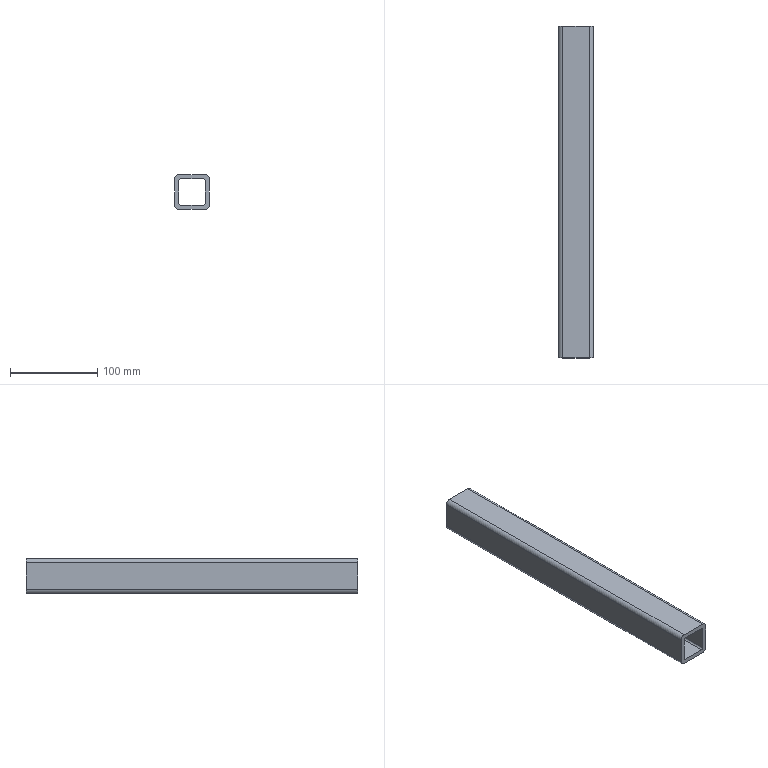Component | SolidWorks | 40-40SquareTube7-1 | 1 solid | 18 faces | box 40 x 380 x 40 mm | volume 259150 mm3 | plane 10 | cylinder 8 | commonest cylinder face diameters 10 x4 4 x4
build123d program:
from build123d import *

# Parameters (mm, degrees)
BOSS_EXTRUDE1_DEPTH = 190


with BuildPart() as part:
    # Sketch1 → Boss-Extrude1 (new, symmetric)
    with BuildSketch(Plane.XY):
        with BuildLine():
            Line((-15, -20), (15, -20))
            ThreePointArc((15, -20), (18.536, -18.536), (20, -15))
            Line((20, -15), (20, 15))
            ThreePointArc((20, 15), (18.536, 18.536), (15, 20))
            Line((15, 20), (-15, 20))
            ThreePointArc((-15, 20), (-18.536, 18.536), (-20, 15))
            Line((-20, 15), (-20, -15))
            ThreePointArc((-20, -15), (-18.536, -18.536), (-15, -20))
        make_face()
        with BuildLine():
            Line((-13, -15), (13, -15))
            ThreePointArc((13, -15), (14.414, -14.414), (15, -13))
            Line((15, -13), (15, 13))
            ThreePointArc((15, 13), (14.414, 14.414), (13, 15))
            Line((13, 15), (-13, 15))
            ThreePointArc((-13, 15), (-14.414, 14.414), (-15, 13))
            Line((-15, 13), (-15, -13))
            ThreePointArc((-15, -13), (-14.414, -14.414), (-13, -15))
        make_face(mode=Mode.SUBTRACT)
    extrude(amount=BOSS_EXTRUDE1_DEPTH, both=True)


solid = part.part

# Placed as in the assembly
solid = solid.moved(Location((17.398, 237.837, 160), (90, 0, 0)))
STEP:
#1=CARTESIAN_POINT('',(1.472,16.844,5.709));
#2=VERTEX_POINT('',#1);
#3=CARTESIAN_POINT('',(1.276,16.844,5.512));
#4=VERTEX_POINT('',#3);
#5=CARTESIAN_POINT('',(1.276,16.844,5.709));
#6=DIRECTION('',(0.,1.,0.));
#7=DIRECTION('',(0.,0.,-1.));
#8=AXIS2_PLACEMENT_3D('',#5,#6,#7);
#9=CIRCLE('',#8,0.1969);
#10=EDGE_CURVE('',#2,#4,#9,.T.);
#11=ORIENTED_EDGE('',*,*,#10,.T.);
#12=CARTESIAN_POINT('',(0.09441,16.844,5.512));
#13=VERTEX_POINT('',#12);
#14=CARTESIAN_POINT('',(1.276,16.844,5.512));
#15=DIRECTION('',(-1.,0.,0.));
#16=VECTOR('',#15,39.37);
#17=LINE('',#14,#16);
#18=EDGE_CURVE('',#4,#13,#17,.T.);
#19=ORIENTED_EDGE('',*,*,#18,.T.);
#20=CARTESIAN_POINT('',(-0.1024,16.844,5.709));
#21=VERTEX_POINT('',#20);
#22=CARTESIAN_POINT('',(0.09441,16.844,5.709));
#23=DIRECTION('',(0.,1.,0.));
#24=DIRECTION('',(0.,0.,1.));
#25=AXIS2_PLACEMENT_3D('',#22,#23,#24);
#26=CIRCLE('',#25,0.1969);
#27=EDGE_CURVE('',#13,#21,#26,.T.);
#28=ORIENTED_EDGE('',*,*,#27,.T.);
#29=CARTESIAN_POINT('',(-0.1024,16.844,6.89));
#30=VERTEX_POINT('',#29);
#31=CARTESIAN_POINT('',(-0.1024,16.844,6.89));
#32=DIRECTION('',(0.,-0.,1.));
#33=VECTOR('',#32,39.37);
#34=LINE('',#31,#33);
#35=EDGE_CURVE('',#21,#30,#34,.T.);
#36=ORIENTED_EDGE('',*,*,#35,.T.);
#37=CARTESIAN_POINT('',(0.09441,16.844,7.087));
#38=VERTEX_POINT('',#37);
#39=CARTESIAN_POINT('',(0.09441,16.844,6.89));
#40=DIRECTION('',(0.,1.,0.));
#41=DIRECTION('',(0.,0.,1.));
#42=AXIS2_PLACEMENT_3D('',#39,#40,#41);
#43=CIRCLE('',#42,0.1969);
#44=EDGE_CURVE('',#30,#38,#43,.T.);
#45=ORIENTED_EDGE('',*,*,#44,.T.);
#46=CARTESIAN_POINT('',(1.276,16.844,7.087));
#47=VERTEX_POINT('',#46);
#48=CARTESIAN_POINT('',(1.276,16.844,7.087));
#49=DIRECTION('',(1.,-0.,0.));
#50=VECTOR('',#49,39.37);
#51=LINE('',#48,#50);
#52=EDGE_CURVE('',#38,#47,#51,.T.);
#53=ORIENTED_EDGE('',*,*,#52,.T.);
#54=CARTESIAN_POINT('',(1.472,16.844,6.89));
#55=VERTEX_POINT('',#54);
#56=CARTESIAN_POINT('',(1.276,16.844,6.89));
#57=DIRECTION('',(0.,1.,0.));
#58=DIRECTION('',(0.,0.,1.));
#59=AXIS2_PLACEMENT_3D('',#56,#57,#58);
#60=CIRCLE('',#59,0.1969);
#61=EDGE_CURVE('',#47,#55,#60,.T.);
#62=ORIENTED_EDGE('',*,*,#61,.T.);
#63=CARTESIAN_POINT('',(1.472,16.844,6.89));
#64=DIRECTION('',(0.,0.,-1.));
#65=VECTOR('',#64,39.37);
#66=LINE('',#63,#65);
#67=EDGE_CURVE('',#55,#2,#66,.T.);
#68=ORIENTED_EDGE('',*,*,#67,.T.);
#69=EDGE_LOOP('',(#11,#19,#28,#36,#45,#53,#62,#68));
#70=FACE_OUTER_BOUND('',#69,.T.);
#71=CARTESIAN_POINT('',(1.197,16.844,5.709));
#72=VERTEX_POINT('',#71);
#73=CARTESIAN_POINT('',(0.1732,16.844,5.709));
#74=VERTEX_POINT('',#73);
#75=CARTESIAN_POINT('',(1.197,16.844,5.709));
#76=DIRECTION('',(-1.,0.,0.));
#77=VECTOR('',#76,39.37);
#78=LINE('',#75,#77);
#79=EDGE_CURVE('',#72,#74,#78,.T.);
#80=ORIENTED_EDGE('',*,*,#79,.F.);
#81=CARTESIAN_POINT('',(1.276,16.844,5.787));
#82=VERTEX_POINT('',#81);
#83=CARTESIAN_POINT('',(1.197,16.844,5.787));
#84=DIRECTION('',(0.,1.,0.));
#85=DIRECTION('',(0.,0.,-1.));
#86=AXIS2_PLACEMENT_3D('',#83,#84,#85);
#87=CIRCLE('',#86,0.07874);
#88=EDGE_CURVE('',#82,#72,#87,.T.);
#89=ORIENTED_EDGE('',*,*,#88,.F.);
#90=CARTESIAN_POINT('',(1.276,16.844,6.811));
#91=VERTEX_POINT('',#90);
#92=CARTESIAN_POINT('',(1.276,16.844,6.811));
#93=DIRECTION('',(0.,0.,-1.));
#94=VECTOR('',#93,39.37);
#95=LINE('',#92,#94);
#96=EDGE_CURVE('',#91,#82,#95,.T.);
#97=ORIENTED_EDGE('',*,*,#96,.F.);
#98=CARTESIAN_POINT('',(1.197,16.844,6.89));
#99=VERTEX_POINT('',#98);
#100=CARTESIAN_POINT('',(1.197,16.844,6.811));
#101=DIRECTION('',(0.,1.,0.));
#102=DIRECTION('',(0.,0.,1.));
#103=AXIS2_PLACEMENT_3D('',#100,#101,#102);
#104=CIRCLE('',#103,0.07874);
#105=EDGE_CURVE('',#99,#91,#104,.T.);
#106=ORIENTED_EDGE('',*,*,#105,.F.);
#107=CARTESIAN_POINT('',(0.1732,16.844,6.89));
#108=VERTEX_POINT('',#107);
#109=CARTESIAN_POINT('',(1.197,16.844,6.89));
#110=DIRECTION('',(1.,-0.,-0.));
#111=VECTOR('',#110,39.37);
#112=LINE('',#109,#111);
#113=EDGE_CURVE('',#108,#99,#112,.T.);
#114=ORIENTED_EDGE('',*,*,#113,.F.);
#115=CARTESIAN_POINT('',(0.09441,16.844,6.811));
#116=VERTEX_POINT('',#115);
#117=CARTESIAN_POINT('',(0.1732,16.844,6.811));
#118=DIRECTION('',(0.,1.,0.));
#119=DIRECTION('',(0.,0.,1.));
#120=AXIS2_PLACEMENT_3D('',#117,#118,#119);
#121=CIRCLE('',#120,0.07874);
#122=EDGE_CURVE('',#116,#108,#121,.T.);
#123=ORIENTED_EDGE('',*,*,#122,.F.);
#124=CARTESIAN_POINT('',(0.09441,16.844,5.787));
#125=VERTEX_POINT('',#124);
#126=CARTESIAN_POINT('',(0.09441,16.844,6.811));
#127=DIRECTION('',(0.,-0.,1.));
#128=VECTOR('',#127,39.37);
#129=LINE('',#126,#128);
#130=EDGE_CURVE('',#125,#116,#129,.T.);
#131=ORIENTED_EDGE('',*,*,#130,.F.);
#132=CARTESIAN_POINT('',(0.1732,16.844,5.787));
#133=DIRECTION('',(0.,1.,0.));
#134=DIRECTION('',(0.,0.,1.));
#135=AXIS2_PLACEMENT_3D('',#132,#133,#134);
#136=CIRCLE('',#135,0.07874);
#137=EDGE_CURVE('',#74,#125,#136,.T.);
#138=ORIENTED_EDGE('',*,*,#137,.F.);
#139=EDGE_LOOP('',(#80,#89,#97,#106,#114,#123,#131,#138));
#140=FACE_BOUND('',#139,.T.);
#141=CARTESIAN_POINT('',(1.276,16.844,5.709));
#142=DIRECTION('',(0.,1.,0.));
#143=DIRECTION('',(0.,0.,-1.));
#144=AXIS2_PLACEMENT_3D('',#141,#142,#143);
#145=PLANE('',#144);
#146=ADVANCED_FACE('',(#70,#140),#145,.T.);
#147=CARTESIAN_POINT('',(1.472,1.883,5.709));
#148=VERTEX_POINT('',#147);
#149=CARTESIAN_POINT('',(1.276,1.883,5.512));
#150=VERTEX_POINT('',#149);
#151=CARTESIAN_POINT('',(1.276,1.883,5.709));
#152=DIRECTION('',(0.,1.,0.));
#153=DIRECTION('',(0.,0.,-1.));
#154=AXIS2_PLACEMENT_3D('',#151,#152,#153);
#155=CIRCLE('',#154,0.1969);
#156=EDGE_CURVE('',#148,#150,#155,.T.);
#157=ORIENTED_EDGE('',*,*,#156,.F.);
#158=CARTESIAN_POINT('',(1.472,1.883,6.89));
#159=VERTEX_POINT('',#158);
#160=CARTESIAN_POINT('',(1.472,1.883,6.89));
#161=DIRECTION('',(0.,0.,-1.));
#162=VECTOR('',#161,39.37);
#163=LINE('',#160,#162);
#164=EDGE_CURVE('',#159,#148,#163,.T.);
#165=ORIENTED_EDGE('',*,*,#164,.F.);
#166=CARTESIAN_POINT('',(1.276,1.883,7.087));
#167=VERTEX_POINT('',#166);
#168=CARTESIAN_POINT('',(1.276,1.883,6.89));
#169=DIRECTION('',(0.,1.,0.));
#170=DIRECTION('',(0.,0.,1.));
#171=AXIS2_PLACEMENT_3D('',#168,#169,#170);
#172=CIRCLE('',#171,0.1969);
#173=EDGE_CURVE('',#167,#159,#172,.T.);
#174=ORIENTED_EDGE('',*,*,#173,.F.);
#175=CARTESIAN_POINT('',(0.09441,1.883,7.087));
#176=VERTEX_POINT('',#175);
#177=CARTESIAN_POINT('',(1.276,1.883,7.087));
#178=DIRECTION('',(1.,-0.,0.));
#179=VECTOR('',#178,39.37);
#180=LINE('',#177,#179);
#181=EDGE_CURVE('',#176,#167,#180,.T.);
#182=ORIENTED_EDGE('',*,*,#181,.F.);
#183=CARTESIAN_POINT('',(-0.1024,1.883,6.89));
#184=VERTEX_POINT('',#183);
#185=CARTESIAN_POINT('',(0.09441,1.883,6.89));
#186=DIRECTION('',(0.,1.,0.));
#187=DIRECTION('',(0.,0.,1.));
#188=AXIS2_PLACEMENT_3D('',#185,#186,#187);
#189=CIRCLE('',#188,0.1969);
#190=EDGE_CURVE('',#184,#176,#189,.T.);
#191=ORIENTED_EDGE('',*,*,#190,.F.);
#192=CARTESIAN_POINT('',(-0.1024,1.883,5.709));
#193=VERTEX_POINT('',#192);
#194=CARTESIAN_POINT('',(-0.1024,1.883,6.89));
#195=DIRECTION('',(0.,-0.,1.));
#196=VECTOR('',#195,39.37);
#197=LINE('',#194,#196);
#198=EDGE_CURVE('',#193,#184,#197,.T.);
#199=ORIENTED_EDGE('',*,*,#198,.F.);
#200=CARTESIAN_POINT('',(0.09441,1.883,5.512));
#201=VERTEX_POINT('',#200);
#202=CARTESIAN_POINT('',(0.09441,1.883,5.709));
#203=DIRECTION('',(0.,1.,0.));
#204=DIRECTION('',(0.,0.,1.));
#205=AXIS2_PLACEMENT_3D('',#202,#203,#204);
#206=CIRCLE('',#205,0.1969);
#207=EDGE_CURVE('',#201,#193,#206,.T.);
#208=ORIENTED_EDGE('',*,*,#207,.F.);
#209=CARTESIAN_POINT('',(1.276,1.883,5.512));
#210=DIRECTION('',(-1.,0.,0.));
#211=VECTOR('',#210,39.37);
#212=LINE('',#209,#211);
#213=EDGE_CURVE('',#150,#201,#212,.T.);
#214=ORIENTED_EDGE('',*,*,#213,.F.);
#215=EDGE_LOOP('',(#157,#165,#174,#182,#191,#199,#208,#214));
#216=FACE_OUTER_BOUND('',#215,.T.);
#217=CARTESIAN_POINT('',(1.276,1.883,5.787));
#218=VERTEX_POINT('',#217);
#219=CARTESIAN_POINT('',(1.197,1.883,5.709));
#220=VERTEX_POINT('',#219);
#221=CARTESIAN_POINT('',(1.197,1.883,5.787));
#222=DIRECTION('',(0.,1.,0.));
#223=DIRECTION('',(0.,0.,-1.));
#224=AXIS2_PLACEMENT_3D('',#221,#222,#223);
#225=CIRCLE('',#224,0.07874);
#226=EDGE_CURVE('',#218,#220,#225,.T.);
#227=ORIENTED_EDGE('',*,*,#226,.T.);
#228=CARTESIAN_POINT('',(0.1732,1.883,5.709));
#229=VERTEX_POINT('',#228);
#230=CARTESIAN_POINT('',(1.197,1.883,5.709));
#231=DIRECTION('',(-1.,0.,0.));
#232=VECTOR('',#231,39.37);
#233=LINE('',#230,#232);
#234=EDGE_CURVE('',#220,#229,#233,.T.);
#235=ORIENTED_EDGE('',*,*,#234,.T.);
#236=CARTESIAN_POINT('',(0.09441,1.883,5.787));
#237=VERTEX_POINT('',#236);
#238=CARTESIAN_POINT('',(0.1732,1.883,5.787));
#239=DIRECTION('',(0.,1.,0.));
#240=DIRECTION('',(0.,0.,1.));
#241=AXIS2_PLACEMENT_3D('',#238,#239,#240);
#242=CIRCLE('',#241,0.07874);
#243=EDGE_CURVE('',#229,#237,#242,.T.);
#244=ORIENTED_EDGE('',*,*,#243,.T.);
#245=CARTESIAN_POINT('',(0.09441,1.883,6.811));
#246=VERTEX_POINT('',#245);
#247=CARTESIAN_POINT('',(0.09441,1.883,6.811));
#248=DIRECTION('',(0.,-0.,1.));
#249=VECTOR('',#248,39.37);
#250=LINE('',#247,#249);
#251=EDGE_CURVE('',#237,#246,#250,.T.);
#252=ORIENTED_EDGE('',*,*,#251,.T.);
#253=CARTESIAN_POINT('',(0.1732,1.883,6.89));
#254=VERTEX_POINT('',#253);
#255=CARTESIAN_POINT('',(0.1732,1.883,6.811));
#256=DIRECTION('',(0.,1.,0.));
#257=DIRECTION('',(0.,0.,1.));
#258=AXIS2_PLACEMENT_3D('',#255,#256,#257);
#259=CIRCLE('',#258,0.07874);
#260=EDGE_CURVE('',#246,#254,#259,.T.);
#261=ORIENTED_EDGE('',*,*,#260,.T.);
#262=CARTESIAN_POINT('',(1.197,1.883,6.89));
#263=VERTEX_POINT('',#262);
#264=CARTESIAN_POINT('',(1.197,1.883,6.89));
#265=DIRECTION('',(1.,-0.,-0.));
#266=VECTOR('',#265,39.37);
#267=LINE('',#264,#266);
#268=EDGE_CURVE('',#254,#263,#267,.T.);
#269=ORIENTED_EDGE('',*,*,#268,.T.);
#270=CARTESIAN_POINT('',(1.276,1.883,6.811));
#271=VERTEX_POINT('',#270);
#272=CARTESIAN_POINT('',(1.197,1.883,6.811));
#273=DIRECTION('',(0.,1.,0.));
#274=DIRECTION('',(0.,0.,1.));
#275=AXIS2_PLACEMENT_3D('',#272,#273,#274);
#276=CIRCLE('',#275,0.07874);
#277=EDGE_CURVE('',#263,#271,#276,.T.);
#278=ORIENTED_EDGE('',*,*,#277,.T.);
#279=CARTESIAN_POINT('',(1.276,1.883,6.811));
#280=DIRECTION('',(0.,0.,-1.));
#281=VECTOR('',#280,39.37);
#282=LINE('',#279,#281);
#283=EDGE_CURVE('',#271,#218,#282,.T.);
#284=ORIENTED_EDGE('',*,*,#283,.T.);
#285=EDGE_LOOP('',(#227,#235,#244,#252,#261,#269,#278,#284));
#286=FACE_BOUND('',#285,.T.);
#287=CARTESIAN_POINT('',(1.276,1.883,5.709));
#288=DIRECTION('',(0.,1.,0.));
#289=DIRECTION('',(0.,0.,-1.));
#290=AXIS2_PLACEMENT_3D('',#287,#288,#289);
#291=PLANE('',#290);
#292=ADVANCED_FACE('',(#216,#286),#291,.F.);
#293=ORIENTED_EDGE('',*,*,#156,.T.);
#294=CARTESIAN_POINT('',(1.276,16.844,5.512));
#295=DIRECTION('',(-0.,-1.,-0.));
#296=VECTOR('',#295,39.37);
#297=LINE('',#294,#296);
#298=EDGE_CURVE('',#4,#150,#297,.T.);
#299=ORIENTED_EDGE('',*,*,#298,.F.);
#300=ORIENTED_EDGE('',*,*,#10,.F.);
#301=CARTESIAN_POINT('',(1.472,16.844,5.709));
#302=DIRECTION('',(-0.,-1.,-0.));
#303=VECTOR('',#302,39.37);
#304=LINE('',#301,#303);
#305=EDGE_CURVE('',#2,#148,#304,.T.);
#306=ORIENTED_EDGE('',*,*,#305,.T.);
#307=EDGE_LOOP('',(#293,#299,#300,#306));
#308=FACE_OUTER_BOUND('',#307,.T.);
#309=CARTESIAN_POINT('',(1.276,16.844,5.709));
#310=DIRECTION('',(-0.,-1.,-0.));
#311=DIRECTION('',(0.,0.,1.));
#312=AXIS2_PLACEMENT_3D('',#309,#310,#311);
#313=CYLINDRICAL_SURFACE('',#312,0.1969);
#314=ADVANCED_FACE('',(#308),#313,.T.);
#315=ORIENTED_EDGE('',*,*,#213,.T.);
#316=CARTESIAN_POINT('',(0.09441,16.844,5.512));
#317=DIRECTION('',(-0.,-1.,-0.));
#318=VECTOR('',#317,39.37);
#319=LINE('',#316,#318);
#320=EDGE_CURVE('',#13,#201,#319,.T.);
#321=ORIENTED_EDGE('',*,*,#320,.F.);
#322=ORIENTED_EDGE('',*,*,#18,.F.);
#323=ORIENTED_EDGE('',*,*,#298,.T.);
#324=EDGE_LOOP('',(#315,#321,#322,#323));
#325=FACE_OUTER_BOUND('',#324,.T.);
#326=CARTESIAN_POINT('',(1.276,16.844,5.512));
#327=DIRECTION('',(0.,-0.,1.));
#328=DIRECTION('',(0.,1.,0.));
#329=AXIS2_PLACEMENT_3D('',#326,#327,#328);
#330=PLANE('',#329);
#331=ADVANCED_FACE('',(#325),#330,.F.);
#332=ORIENTED_EDGE('',*,*,#207,.T.);
#333=CARTESIAN_POINT('',(-0.1024,16.844,5.709));
#334=DIRECTION('',(-0.,-1.,-0.));
#335=VECTOR('',#334,39.37);
#336=LINE('',#333,#335);
#337=EDGE_CURVE('',#21,#193,#336,.T.);
#338=ORIENTED_EDGE('',*,*,#337,.F.);
#339=ORIENTED_EDGE('',*,*,#27,.F.);
#340=ORIENTED_EDGE('',*,*,#320,.T.);
#341=EDGE_LOOP('',(#332,#338,#339,#340));
#342=FACE_OUTER_BOUND('',#341,.T.);
#343=CARTESIAN_POINT('',(0.09441,16.844,5.709));
#344=DIRECTION('',(-0.,-1.,-0.));
#345=DIRECTION('',(0.,0.,1.));
#346=AXIS2_PLACEMENT_3D('',#343,#344,#345);
#347=CYLINDRICAL_SURFACE('',#346,0.1969);
#348=ADVANCED_FACE('',(#342),#347,.T.);
#349=ORIENTED_EDGE('',*,*,#198,.T.);
#350=CARTESIAN_POINT('',(-0.1024,16.844,6.89));
#351=DIRECTION('',(-0.,-1.,-0.));
#352=VECTOR('',#351,39.37);
#353=LINE('',#350,#352);
#354=EDGE_CURVE('',#30,#184,#353,.T.);
#355=ORIENTED_EDGE('',*,*,#354,.F.);
#356=ORIENTED_EDGE('',*,*,#35,.F.);
#357=ORIENTED_EDGE('',*,*,#337,.T.);
#358=EDGE_LOOP('',(#349,#355,#356,#357));
#359=FACE_OUTER_BOUND('',#358,.T.);
#360=CARTESIAN_POINT('',(-0.1024,16.844,6.89));
#361=DIRECTION('',(1.,-0.,-0.));
#362=DIRECTION('',(-0.,-1.,-0.));
#363=AXIS2_PLACEMENT_3D('',#360,#361,#362);
#364=PLANE('',#363);
#365=ADVANCED_FACE('',(#359),#364,.F.);
#366=ORIENTED_EDGE('',*,*,#190,.T.);
#367=CARTESIAN_POINT('',(0.09441,16.844,7.087));
#368=DIRECTION('',(-0.,-1.,-0.));
#369=VECTOR('',#368,39.37);
#370=LINE('',#367,#369);
#371=EDGE_CURVE('',#38,#176,#370,.T.);
#372=ORIENTED_EDGE('',*,*,#371,.F.);
#373=ORIENTED_EDGE('',*,*,#44,.F.);
#374=ORIENTED_EDGE('',*,*,#354,.T.);
#375=EDGE_LOOP('',(#366,#372,#373,#374));
#376=FACE_OUTER_BOUND('',#375,.T.);
#377=CARTESIAN_POINT('',(0.09441,16.844,6.89));
#378=DIRECTION('',(-0.,-1.,-0.));
#379=DIRECTION('',(0.,0.,1.));
#380=AXIS2_PLACEMENT_3D('',#377,#378,#379);
#381=CYLINDRICAL_SURFACE('',#380,0.1969);
#382=ADVANCED_FACE('',(#376),#381,.T.);
#383=ORIENTED_EDGE('',*,*,#181,.T.);
#384=CARTESIAN_POINT('',(1.276,16.844,7.087));
#385=DIRECTION('',(-0.,-1.,-0.));
#386=VECTOR('',#385,39.37);
#387=LINE('',#384,#386);
#388=EDGE_CURVE('',#47,#167,#387,.T.);
#389=ORIENTED_EDGE('',*,*,#388,.F.);
#390=ORIENTED_EDGE('',*,*,#52,.F.);
#391=ORIENTED_EDGE('',*,*,#371,.T.);
#392=EDGE_LOOP('',(#383,#389,#390,#391));
#393=FACE_OUTER_BOUND('',#392,.T.);
#394=CARTESIAN_POINT('',(1.276,16.844,7.087));
#395=DIRECTION('',(0.,0.,-1.));
#396=DIRECTION('',(-1.,0.,-0.));
#397=AXIS2_PLACEMENT_3D('',#394,#395,#396);
#398=PLANE('',#397);
#399=ADVANCED_FACE('',(#393),#398,.F.);
#400=ORIENTED_EDGE('',*,*,#173,.T.);
#401=CARTESIAN_POINT('',(1.472,16.844,6.89));
#402=DIRECTION('',(-0.,-1.,-0.));
#403=VECTOR('',#402,39.37);
#404=LINE('',#401,#403);
#405=EDGE_CURVE('',#55,#159,#404,.T.);
#406=ORIENTED_EDGE('',*,*,#405,.F.);
#407=ORIENTED_EDGE('',*,*,#61,.F.);
#408=ORIENTED_EDGE('',*,*,#388,.T.);
#409=EDGE_LOOP('',(#400,#406,#407,#408));
#410=FACE_OUTER_BOUND('',#409,.T.);
#411=CARTESIAN_POINT('',(1.276,16.844,6.89));
#412=DIRECTION('',(-0.,-1.,-0.));
#413=DIRECTION('',(0.,0.,1.));
#414=AXIS2_PLACEMENT_3D('',#411,#412,#413);
#415=CYLINDRICAL_SURFACE('',#414,0.1969);
#416=ADVANCED_FACE('',(#410),#415,.T.);
#417=ORIENTED_EDGE('',*,*,#164,.T.);
#418=ORIENTED_EDGE('',*,*,#305,.F.);
#419=ORIENTED_EDGE('',*,*,#67,.F.);
#420=ORIENTED_EDGE('',*,*,#405,.T.);
#421=EDGE_LOOP('',(#417,#418,#419,#420));
#422=FACE_OUTER_BOUND('',#421,.T.);
#423=CARTESIAN_POINT('',(1.472,16.844,6.89));
#424=DIRECTION('',(-1.,0.,0.));
#425=DIRECTION('',(0.,1.,0.));
#426=AXIS2_PLACEMENT_3D('',#423,#424,#425);
#427=PLANE('',#426);
#428=ADVANCED_FACE('',(#422),#427,.F.);
#429=ORIENTED_EDGE('',*,*,#226,.F.);
#430=CARTESIAN_POINT('',(1.276,16.844,5.787));
#431=DIRECTION('',(-0.,-1.,-0.));
#432=VECTOR('',#431,39.37);
#433=LINE('',#430,#432);
#434=EDGE_CURVE('',#82,#218,#433,.T.);
#435=ORIENTED_EDGE('',*,*,#434,.F.);
#436=ORIENTED_EDGE('',*,*,#88,.T.);
#437=CARTESIAN_POINT('',(1.197,16.844,5.709));
#438=DIRECTION('',(-0.,-1.,-0.));
#439=VECTOR('',#438,39.37);
#440=LINE('',#437,#439);
#441=EDGE_CURVE('',#72,#220,#440,.T.);
#442=ORIENTED_EDGE('',*,*,#441,.T.);
#443=EDGE_LOOP('',(#429,#435,#436,#442));
#444=FACE_OUTER_BOUND('',#443,.T.);
#445=CARTESIAN_POINT('',(1.197,16.844,5.787));
#446=DIRECTION('',(-0.,-1.,-0.));
#447=DIRECTION('',(0.,0.,1.));
#448=AXIS2_PLACEMENT_3D('',#445,#446,#447);
#449=CYLINDRICAL_SURFACE('',#448,0.07874);
#450=ADVANCED_FACE('',(#444),#449,.F.);
#451=ORIENTED_EDGE('',*,*,#234,.F.);
#452=ORIENTED_EDGE('',*,*,#441,.F.);
#453=ORIENTED_EDGE('',*,*,#79,.T.);
#454=CARTESIAN_POINT('',(0.1732,16.844,5.709));
#455=DIRECTION('',(-0.,-1.,-0.));
#456=VECTOR('',#455,39.37);
#457=LINE('',#454,#456);
#458=EDGE_CURVE('',#74,#229,#457,.T.);
#459=ORIENTED_EDGE('',*,*,#458,.T.);
#460=EDGE_LOOP('',(#451,#452,#453,#459));
#461=FACE_OUTER_BOUND('',#460,.T.);
#462=CARTESIAN_POINT('',(1.197,16.844,5.709));
#463=DIRECTION('',(0.,-0.,1.));
#464=DIRECTION('',(0.,1.,0.));
#465=AXIS2_PLACEMENT_3D('',#462,#463,#464);
#466=PLANE('',#465);
#467=ADVANCED_FACE('',(#461),#466,.T.);
#468=ORIENTED_EDGE('',*,*,#243,.F.);
#469=ORIENTED_EDGE('',*,*,#458,.F.);
#470=ORIENTED_EDGE('',*,*,#137,.T.);
#471=CARTESIAN_POINT('',(0.09441,16.844,5.787));
#472=DIRECTION('',(-0.,-1.,-0.));
#473=VECTOR('',#472,39.37);
#474=LINE('',#471,#473);
#475=EDGE_CURVE('',#125,#237,#474,.T.);
#476=ORIENTED_EDGE('',*,*,#475,.T.);
#477=EDGE_LOOP('',(#468,#469,#470,#476));
#478=FACE_OUTER_BOUND('',#477,.T.);
#479=CARTESIAN_POINT('',(0.1732,16.844,5.787));
#480=DIRECTION('',(-0.,-1.,-0.));
#481=DIRECTION('',(0.,0.,1.));
#482=AXIS2_PLACEMENT_3D('',#479,#480,#481);
#483=CYLINDRICAL_SURFACE('',#482,0.07874);
#484=ADVANCED_FACE('',(#478),#483,.F.);
#485=ORIENTED_EDGE('',*,*,#251,.F.);
#486=ORIENTED_EDGE('',*,*,#475,.F.);
#487=ORIENTED_EDGE('',*,*,#130,.T.);
#488=CARTESIAN_POINT('',(0.09441,16.844,6.811));
#489=DIRECTION('',(-0.,-1.,-0.));
#490=VECTOR('',#489,39.37);
#491=LINE('',#488,#490);
#492=EDGE_CURVE('',#116,#246,#491,.T.);
#493=ORIENTED_EDGE('',*,*,#492,.T.);
#494=EDGE_LOOP('',(#485,#486,#487,#493));
#495=FACE_OUTER_BOUND('',#494,.T.);
#496=CARTESIAN_POINT('',(0.09441,16.844,6.811));
#497=DIRECTION('',(1.,-0.,-0.));
#498=DIRECTION('',(-0.,-1.,-0.));
#499=AXIS2_PLACEMENT_3D('',#496,#497,#498);
#500=PLANE('',#499);
#501=ADVANCED_FACE('',(#495),#500,.T.);
#502=ORIENTED_EDGE('',*,*,#260,.F.);
#503=ORIENTED_EDGE('',*,*,#492,.F.);
#504=ORIENTED_EDGE('',*,*,#122,.T.);
#505=CARTESIAN_POINT('',(0.1732,16.844,6.89));
#506=DIRECTION('',(-0.,-1.,-0.));
#507=VECTOR('',#506,39.37);
#508=LINE('',#505,#507);
#509=EDGE_CURVE('',#108,#254,#508,.T.);
#510=ORIENTED_EDGE('',*,*,#509,.T.);
#511=EDGE_LOOP('',(#502,#503,#504,#510));
#512=FACE_OUTER_BOUND('',#511,.T.);
#513=CARTESIAN_POINT('',(0.1732,16.844,6.811));
#514=DIRECTION('',(-0.,-1.,-0.));
#515=DIRECTION('',(0.,0.,1.));
#516=AXIS2_PLACEMENT_3D('',#513,#514,#515);
#517=CYLINDRICAL_SURFACE('',#516,0.07874);
#518=ADVANCED_FACE('',(#512),#517,.F.);
#519=ORIENTED_EDGE('',*,*,#268,.F.);
#520=ORIENTED_EDGE('',*,*,#509,.F.);
#521=ORIENTED_EDGE('',*,*,#113,.T.);
#522=CARTESIAN_POINT('',(1.197,16.844,6.89));
#523=DIRECTION('',(-0.,-1.,-0.));
#524=VECTOR('',#523,39.37);
#525=LINE('',#522,#524);
#526=EDGE_CURVE('',#99,#263,#525,.T.);
#527=ORIENTED_EDGE('',*,*,#526,.T.);
#528=EDGE_LOOP('',(#519,#520,#521,#527));
#529=FACE_OUTER_BOUND('',#528,.T.);
#530=CARTESIAN_POINT('',(1.197,16.844,6.89));
#531=DIRECTION('',(0.,0.,-1.));
#532=DIRECTION('',(-0.,-1.,-0.));
#533=AXIS2_PLACEMENT_3D('',#530,#531,#532);
#534=PLANE('',#533);
#535=ADVANCED_FACE('',(#529),#534,.T.);
#536=ORIENTED_EDGE('',*,*,#277,.F.);
#537=ORIENTED_EDGE('',*,*,#526,.F.);
#538=ORIENTED_EDGE('',*,*,#105,.T.);
#539=CARTESIAN_POINT('',(1.276,16.844,6.811));
#540=DIRECTION('',(-0.,-1.,-0.));
#541=VECTOR('',#540,39.37);
#542=LINE('',#539,#541);
#543=EDGE_CURVE('',#91,#271,#542,.T.);
#544=ORIENTED_EDGE('',*,*,#543,.T.);
#545=EDGE_LOOP('',(#536,#537,#538,#544));
#546=FACE_OUTER_BOUND('',#545,.T.);
#547=CARTESIAN_POINT('',(1.197,16.844,6.811));
#548=DIRECTION('',(-0.,-1.,-0.));
#549=DIRECTION('',(0.,0.,1.));
#550=AXIS2_PLACEMENT_3D('',#547,#548,#549);
#551=CYLINDRICAL_SURFACE('',#550,0.07874);
#552=ADVANCED_FACE('',(#546),#551,.F.);
#553=ORIENTED_EDGE('',*,*,#283,.F.);
#554=ORIENTED_EDGE('',*,*,#543,.F.);
#555=ORIENTED_EDGE('',*,*,#96,.T.);
#556=ORIENTED_EDGE('',*,*,#434,.T.);
#557=EDGE_LOOP('',(#553,#554,#555,#556));
#558=FACE_OUTER_BOUND('',#557,.T.);
#559=CARTESIAN_POINT('',(1.276,16.844,6.811));
#560=DIRECTION('',(-1.,0.,0.));
#561=DIRECTION('',(0.,1.,0.));
#562=AXIS2_PLACEMENT_3D('',#559,#560,#561);
#563=PLANE('',#562);
#564=ADVANCED_FACE('',(#558),#563,.T.);
#565=CLOSED_SHELL('',(#146,#292,#314,#331,#348,#365,#382,#399,#416,#428,#450,#467,#484,#501,#518,#535,#552,#564));
#566=MANIFOLD_SOLID_BREP('',#565);
#567=CARTESIAN_POINT('',(0.,0.,0.));
#568=DIRECTION('',(0.,0.,1.));
#569=DIRECTION('',(1.,0.,0.));
#570=AXIS2_PLACEMENT_3D('',#567,#568,#569);
#571=(LENGTH_UNIT()NAMED_UNIT(*)SI_UNIT($,.METRE.));
#572=LENGTH_MEASURE_WITH_UNIT(LENGTH_MEASURE(0.0254),#571);
#573=DIMENSIONAL_EXPONENTS(1.,0.,0.,0.,0.,0.,0.);
#574=(CONVERSION_BASED_UNIT('',#572)LENGTH_UNIT()NAMED_UNIT(#573));
#575=UNCERTAINTY_MEASURE_WITH_UNIT(LENGTH_MEASURE(0.00001),#574,'','');
#576=(NAMED_UNIT(*)PLANE_ANGLE_UNIT()SI_UNIT($,.RADIAN.));
#577=(NAMED_UNIT(*)SI_UNIT($,.STERADIAN.)SOLID_ANGLE_UNIT());
#578=(GEOMETRIC_REPRESENTATION_CONTEXT(3)GLOBAL_UNCERTAINTY_ASSIGNED_CONTEXT((#575))GLOBAL_UNIT_ASSIGNED_CONTEXT((#574,#576,#577))REPRESENTATION_CONTEXT('',''));
#579=ADVANCED_BREP_SHAPE_REPRESENTATION('',(#566,#570),#578);
#580=COLOUR_RGB('',0.7922,0.8196,0.9333);
#581=FILL_AREA_STYLE_COLOUR('',#580);
#582=FILL_AREA_STYLE('',(#581));
#583=SURFACE_STYLE_FILL_AREA(#582);
#584=SURFACE_SIDE_STYLE('',(#583));
#585=SURFACE_STYLE_USAGE(.BOTH.,#584);
#586=PRESENTATION_STYLE_ASSIGNMENT((#585));
#587=STYLED_ITEM('',(#586),#566);
#588=PRESENTATION_LAYER_ASSIGNMENT('','',(#587));
#589=(LENGTH_UNIT()NAMED_UNIT(*)SI_UNIT($,.METRE.));
#590=LENGTH_MEASURE_WITH_UNIT(LENGTH_MEASURE(0.0254),#589);
#591=DIMENSIONAL_EXPONENTS(1.,0.,0.,0.,0.,0.,0.);
#592=(CONVERSION_BASED_UNIT('',#590)LENGTH_UNIT()NAMED_UNIT(#591));
#593=UNCERTAINTY_MEASURE_WITH_UNIT(LENGTH_MEASURE(0.00001),#592,'','');
#594=(NAMED_UNIT(*)PLANE_ANGLE_UNIT()SI_UNIT($,.RADIAN.));
#595=(NAMED_UNIT(*)SI_UNIT($,.STERADIAN.)SOLID_ANGLE_UNIT());
#596=(GEOMETRIC_REPRESENTATION_CONTEXT(3)GLOBAL_UNCERTAINTY_ASSIGNED_CONTEXT((#593))GLOBAL_UNIT_ASSIGNED_CONTEXT((#592,#594,#595))REPRESENTATION_CONTEXT('',''));
#597=MECHANICAL_DESIGN_GEOMETRIC_PRESENTATION_REPRESENTATION('',(#587),#596);